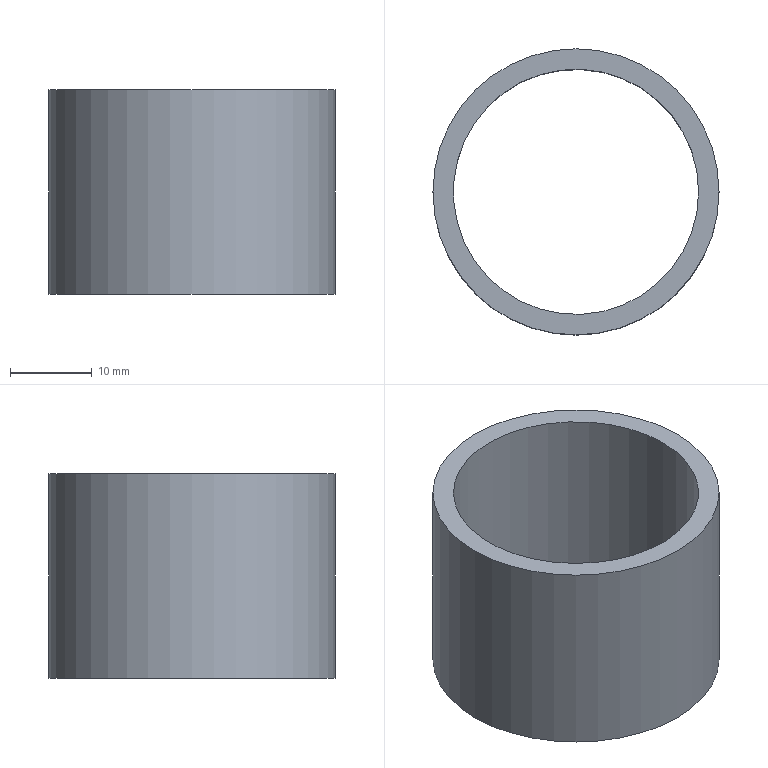Component | NX | SLEEVE | 1 solid | 4 faces | box 35 x 35 x 25 mm | volume 6381 mm3 | cylinder 2 | plane 2 | commonest cylinder face diameters 35 x1 30 x1
STEP:
#1=CARTESIAN_POINT('',(0.,0.,0.));
#2=DIRECTION('',(0.,0.,1.));
#3=DIRECTION('',(1.,0.,0.));
#4=AXIS2_PLACEMENT_3D('',#1,#2,#3);
#5=CARTESIAN_POINT('',(141.5,0.,100.));
#6=VERTEX_POINT('',#5);
#7=CARTESIAN_POINT('',(124.,0.,100.));
#8=DIRECTION('',(0.,0.,1.));
#9=DIRECTION('',(1.,0.,0.));
#10=AXIS2_PLACEMENT_3D('',#7,#8,#9);
#11=CIRCLE('',#10,17.5);
#12=CARTESIAN_POINT('',(124.,0.,100.));
#13=DIRECTION('',(0.,0.,-1.));
#14=DIRECTION('',(-1.,0.,0.));
#15=AXIS2_PLACEMENT_3D('',#12,#13,#14);
#16=CYLINDRICAL_SURFACE('',#15,17.5);
#17=CARTESIAN_POINT('',(9.425,0.));
#18=DIRECTION('',(-1.,0.));
#19=VECTOR('',#18,1.);
#20=LINE('',#17,#19);
#21=(GEOMETRIC_REPRESENTATION_CONTEXT(2)PARAMETRIC_REPRESENTATION_CONTEXT()REPRESENTATION_CONTEXT('',''));
#22=DEFINITIONAL_REPRESENTATION('',(#20),#21);
#23=PCURVE('',#16,#22);
#24=CARTESIAN_POINT('',(124.,0.,100.));
#25=DIRECTION('',(0.,0.,1.));
#26=DIRECTION('',(1.,0.,0.));
#27=AXIS2_PLACEMENT_3D('',#24,#25,#26);
#28=PLANE('',#27);
#29=CARTESIAN_POINT('',(0.,0.));
#30=DIRECTION('',(1.,0.));
#31=AXIS2_PLACEMENT_2D('',#29,#30);
#32=CIRCLE('',#31,17.5);
#33=(GEOMETRIC_REPRESENTATION_CONTEXT(2)PARAMETRIC_REPRESENTATION_CONTEXT()REPRESENTATION_CONTEXT('',''));
#34=DEFINITIONAL_REPRESENTATION('',(#32),#33);
#35=PCURVE('',#28,#34);
#36=SURFACE_CURVE('',#11,(#23,#35),.PCURVE_S1.);
#37=EDGE_CURVE('',#6,#6,#36,.T.);
#38=ORIENTED_EDGE('',*,*,#37,.F.);
#39=CARTESIAN_POINT('',(141.5,0.,75.));
#40=VERTEX_POINT('',#39);
#41=CARTESIAN_POINT('',(141.5,0.,100.));
#42=CARTESIAN_POINT('',(141.5,0.,75.));
#43=B_SPLINE_CURVE_WITH_KNOTS('',1,(#41,#42),.UNSPECIFIED.,.F.,.F.,(2,2),(0.,25.),.PIECEWISE_BEZIER_KNOTS.);
#44=CARTESIAN_POINT('',(9.425,0.));
#45=DIRECTION('',(0.,1.));
#46=VECTOR('',#45,1.);
#47=LINE('',#44,#46);
#48=(GEOMETRIC_REPRESENTATION_CONTEXT(2)PARAMETRIC_REPRESENTATION_CONTEXT()REPRESENTATION_CONTEXT('',''));
#49=DEFINITIONAL_REPRESENTATION('',(#47),#48);
#50=PCURVE('',#16,#49);
#51=CARTESIAN_POINT('',(3.142,0.));
#52=DIRECTION('',(0.,1.));
#53=VECTOR('',#52,1.);
#54=LINE('',#51,#53);
#55=(GEOMETRIC_REPRESENTATION_CONTEXT(2)PARAMETRIC_REPRESENTATION_CONTEXT()REPRESENTATION_CONTEXT('',''));
#56=DEFINITIONAL_REPRESENTATION('',(#54),#55);
#57=PCURVE('',#16,#56);
#58=SEAM_CURVE('',#43,(#50,#57),.PCURVE_S1.);
#59=EDGE_CURVE('',#6,#40,#58,.T.);
#60=ORIENTED_EDGE('',*,*,#59,.T.);
#61=CARTESIAN_POINT('',(124.,0.,75.));
#62=DIRECTION('',(0.,0.,1.));
#63=DIRECTION('',(1.,0.,0.));
#64=AXIS2_PLACEMENT_3D('',#61,#62,#63);
#65=CIRCLE('',#64,17.5);
#66=CARTESIAN_POINT('',(9.425,25.));
#67=DIRECTION('',(-1.,0.));
#68=VECTOR('',#67,1.);
#69=LINE('',#66,#68);
#70=(GEOMETRIC_REPRESENTATION_CONTEXT(2)PARAMETRIC_REPRESENTATION_CONTEXT()REPRESENTATION_CONTEXT('',''));
#71=DEFINITIONAL_REPRESENTATION('',(#69),#70);
#72=PCURVE('',#16,#71);
#73=CARTESIAN_POINT('',(124.,0.,75.));
#74=DIRECTION('',(0.,0.,1.));
#75=DIRECTION('',(1.,0.,0.));
#76=AXIS2_PLACEMENT_3D('',#73,#74,#75);
#77=PLANE('',#76);
#78=CARTESIAN_POINT('',(0.,0.));
#79=DIRECTION('',(1.,0.));
#80=AXIS2_PLACEMENT_2D('',#78,#79);
#81=CIRCLE('',#80,17.5);
#82=(GEOMETRIC_REPRESENTATION_CONTEXT(2)PARAMETRIC_REPRESENTATION_CONTEXT()REPRESENTATION_CONTEXT('',''));
#83=DEFINITIONAL_REPRESENTATION('',(#81),#82);
#84=PCURVE('',#77,#83);
#85=SURFACE_CURVE('',#65,(#72,#84),.PCURVE_S1.);
#86=EDGE_CURVE('',#40,#40,#85,.T.);
#87=ORIENTED_EDGE('',*,*,#86,.T.);
#88=ORIENTED_EDGE('',*,*,#59,.F.);
#89=EDGE_LOOP('',(#38,#60,#87,#88));
#90=FACE_BOUND('',#89,.T.);
#91=ADVANCED_FACE('',(#90),#16,.T.);
#92=CARTESIAN_POINT('',(139.,0.,100.));
#93=VERTEX_POINT('',#92);
#94=CARTESIAN_POINT('',(124.,0.,100.));
#95=DIRECTION('',(0.,0.,1.));
#96=DIRECTION('',(1.,0.,0.));
#97=AXIS2_PLACEMENT_3D('',#94,#95,#96);
#98=CIRCLE('',#97,15.);
#99=CARTESIAN_POINT('',(124.,0.,100.));
#100=DIRECTION('',(0.,0.,-1.));
#101=DIRECTION('',(-1.,0.,0.));
#102=AXIS2_PLACEMENT_3D('',#99,#100,#101);
#103=CYLINDRICAL_SURFACE('',#102,15.);
#104=CARTESIAN_POINT('',(9.425,0.));
#105=DIRECTION('',(-1.,0.));
#106=VECTOR('',#105,1.);
#107=LINE('',#104,#106);
#108=(GEOMETRIC_REPRESENTATION_CONTEXT(2)PARAMETRIC_REPRESENTATION_CONTEXT()REPRESENTATION_CONTEXT('',''));
#109=DEFINITIONAL_REPRESENTATION('',(#107),#108);
#110=PCURVE('',#103,#109);
#111=CARTESIAN_POINT('',(0.,0.));
#112=DIRECTION('',(1.,0.));
#113=AXIS2_PLACEMENT_2D('',#111,#112);
#114=CIRCLE('',#113,15.);
#115=(GEOMETRIC_REPRESENTATION_CONTEXT(2)PARAMETRIC_REPRESENTATION_CONTEXT()REPRESENTATION_CONTEXT('',''));
#116=DEFINITIONAL_REPRESENTATION('',(#114),#115);
#117=PCURVE('',#28,#116);
#118=SURFACE_CURVE('',#98,(#110,#117),.PCURVE_S1.);
#119=EDGE_CURVE('',#93,#93,#118,.T.);
#120=ORIENTED_EDGE('',*,*,#119,.F.);
#121=CARTESIAN_POINT('',(139.,0.,75.));
#122=VERTEX_POINT('',#121);
#123=CARTESIAN_POINT('',(139.,0.,100.));
#124=CARTESIAN_POINT('',(139.,0.,75.));
#125=B_SPLINE_CURVE_WITH_KNOTS('',1,(#123,#124),.UNSPECIFIED.,.F.,.F.,(2,2),(0.,25.),.PIECEWISE_BEZIER_KNOTS.);
#126=CARTESIAN_POINT('',(9.425,0.));
#127=DIRECTION('',(0.,1.));
#128=VECTOR('',#127,1.);
#129=LINE('',#126,#128);
#130=(GEOMETRIC_REPRESENTATION_CONTEXT(2)PARAMETRIC_REPRESENTATION_CONTEXT()REPRESENTATION_CONTEXT('',''));
#131=DEFINITIONAL_REPRESENTATION('',(#129),#130);
#132=PCURVE('',#103,#131);
#133=CARTESIAN_POINT('',(3.142,0.));
#134=DIRECTION('',(0.,1.));
#135=VECTOR('',#134,1.);
#136=LINE('',#133,#135);
#137=(GEOMETRIC_REPRESENTATION_CONTEXT(2)PARAMETRIC_REPRESENTATION_CONTEXT()REPRESENTATION_CONTEXT('',''));
#138=DEFINITIONAL_REPRESENTATION('',(#136),#137);
#139=PCURVE('',#103,#138);
#140=SEAM_CURVE('',#125,(#132,#139),.PCURVE_S1.);
#141=EDGE_CURVE('',#93,#122,#140,.T.);
#142=ORIENTED_EDGE('',*,*,#141,.T.);
#143=CARTESIAN_POINT('',(124.,0.,75.));
#144=DIRECTION('',(0.,0.,1.));
#145=DIRECTION('',(1.,0.,0.));
#146=AXIS2_PLACEMENT_3D('',#143,#144,#145);
#147=CIRCLE('',#146,15.);
#148=CARTESIAN_POINT('',(9.425,25.));
#149=DIRECTION('',(-1.,0.));
#150=VECTOR('',#149,1.);
#151=LINE('',#148,#150);
#152=(GEOMETRIC_REPRESENTATION_CONTEXT(2)PARAMETRIC_REPRESENTATION_CONTEXT()REPRESENTATION_CONTEXT('',''));
#153=DEFINITIONAL_REPRESENTATION('',(#151),#152);
#154=PCURVE('',#103,#153);
#155=CARTESIAN_POINT('',(0.,0.));
#156=DIRECTION('',(1.,0.));
#157=AXIS2_PLACEMENT_2D('',#155,#156);
#158=CIRCLE('',#157,15.);
#159=(GEOMETRIC_REPRESENTATION_CONTEXT(2)PARAMETRIC_REPRESENTATION_CONTEXT()REPRESENTATION_CONTEXT('',''));
#160=DEFINITIONAL_REPRESENTATION('',(#158),#159);
#161=PCURVE('',#77,#160);
#162=SURFACE_CURVE('',#147,(#154,#161),.PCURVE_S1.);
#163=EDGE_CURVE('',#122,#122,#162,.T.);
#164=ORIENTED_EDGE('',*,*,#163,.T.);
#165=ORIENTED_EDGE('',*,*,#141,.F.);
#166=EDGE_LOOP('',(#120,#142,#164,#165));
#167=FACE_BOUND('',#166,.F.);
#168=ADVANCED_FACE('',(#167),#103,.F.);
#169=ORIENTED_EDGE('',*,*,#37,.T.);
#170=EDGE_LOOP('',(#169));
#171=FACE_BOUND('',#170,.T.);
#172=ORIENTED_EDGE('',*,*,#119,.F.);
#173=EDGE_LOOP('',(#172));
#174=FACE_BOUND('',#173,.T.);
#175=ADVANCED_FACE('',(#171,#174),#28,.T.);
#176=ORIENTED_EDGE('',*,*,#86,.F.);
#177=EDGE_LOOP('',(#176));
#178=FACE_BOUND('',#177,.T.);
#179=ORIENTED_EDGE('',*,*,#163,.T.);
#180=EDGE_LOOP('',(#179));
#181=FACE_BOUND('',#180,.T.);
#182=ADVANCED_FACE('',(#178,#181),#77,.F.);
#183=CLOSED_SHELL('',(#91,#168,#175,#182));
#184=MANIFOLD_SOLID_BREP('',#183);
#185=(LENGTH_UNIT()NAMED_UNIT(*)SI_UNIT(.MILLI.,.METRE.));
#186=UNCERTAINTY_MEASURE_WITH_UNIT(LENGTH_MEASURE(0.00001),#185,'','');
#187=(NAMED_UNIT(*)PLANE_ANGLE_UNIT()SI_UNIT($,.RADIAN.));
#188=(NAMED_UNIT(*)SI_UNIT($,.STERADIAN.)SOLID_ANGLE_UNIT());
#189=(GEOMETRIC_REPRESENTATION_CONTEXT(3)GLOBAL_UNCERTAINTY_ASSIGNED_CONTEXT((#186))GLOBAL_UNIT_ASSIGNED_CONTEXT((#185,#187,#188))REPRESENTATION_CONTEXT('',''));
#190=ADVANCED_BREP_SHAPE_REPRESENTATION('',(#4,#184),#189);